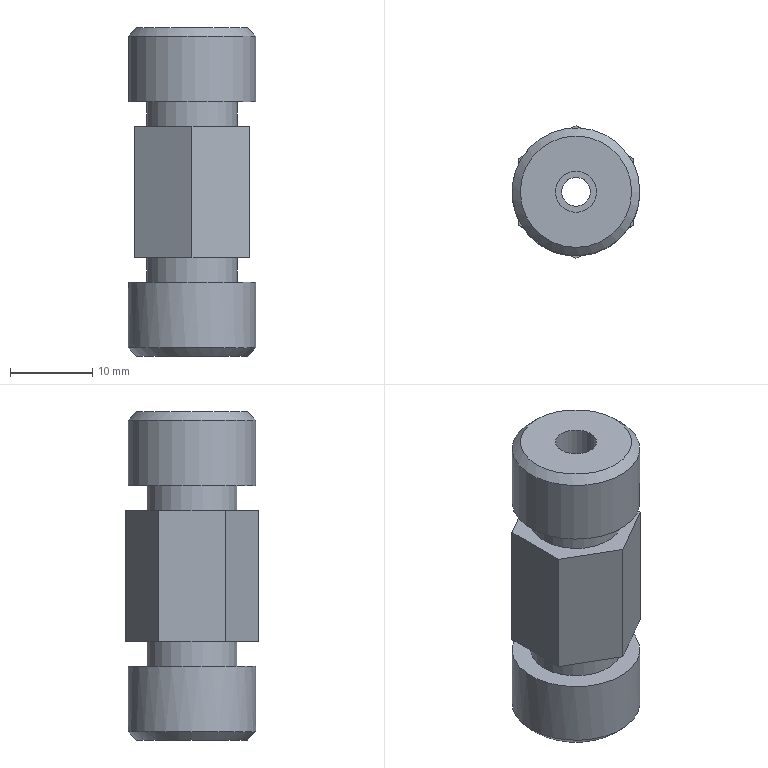Component | NX | DXF_01_VALVE_BODY | 1 solid | 26 faces | volume 5304 mm3 | plane 14 | cylinder 8 | cone 4 | commonest cylinder face diameters 15.568 x2 11 x2 5 x1 7.785 x1 3.5 x1 6.5 x1